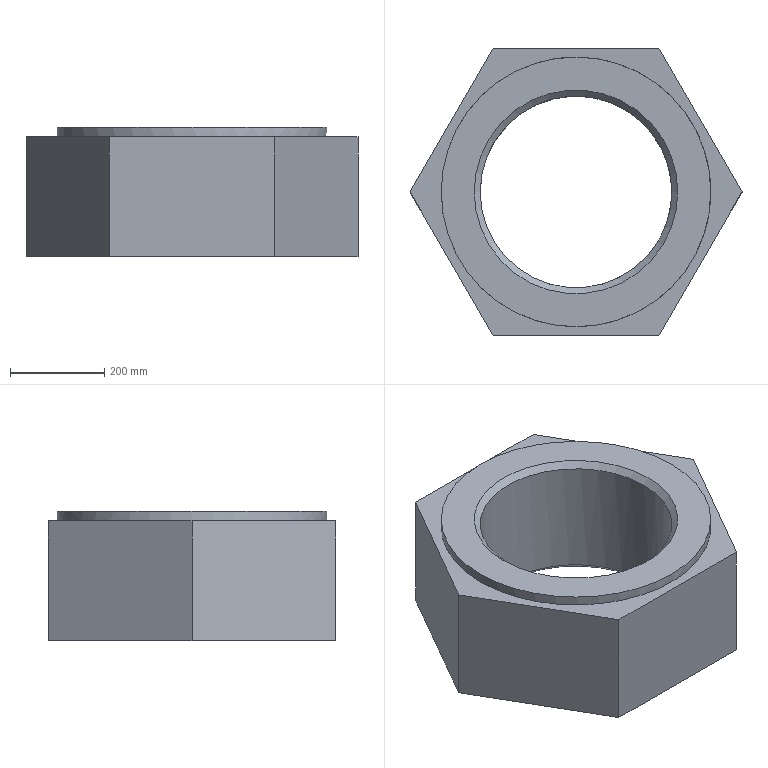Component | NX | 13 | 1 solid | 13 faces | volume 51161980 mm3 | plane 9 | cylinder 2 | cone 2 | commonest cylinder face diameters 571.5 x1 406.4 x1